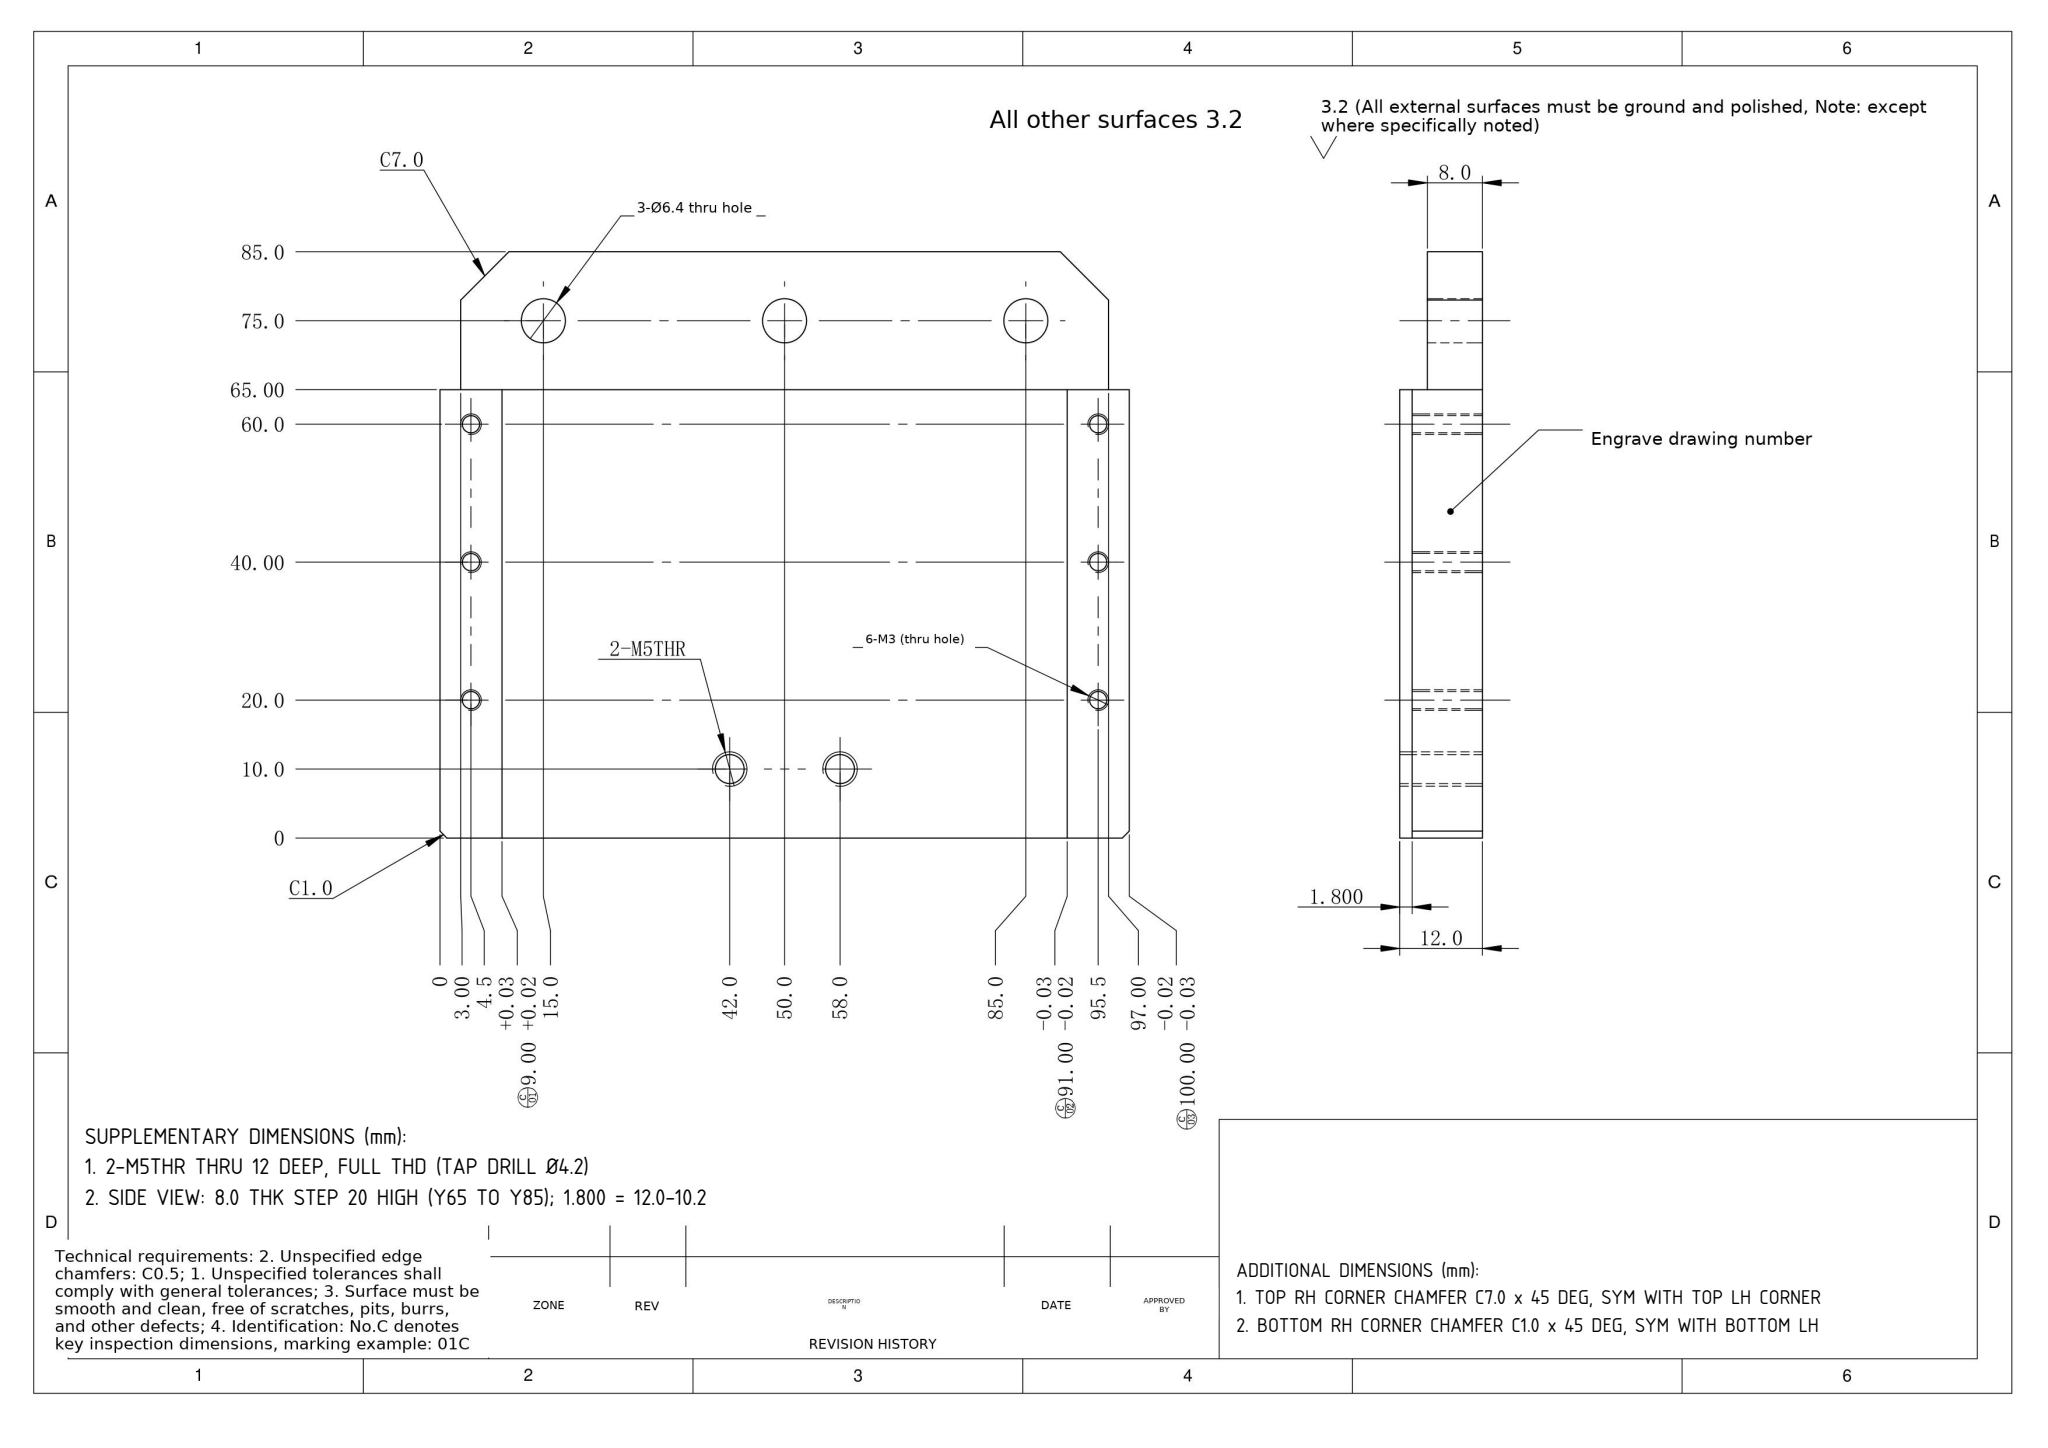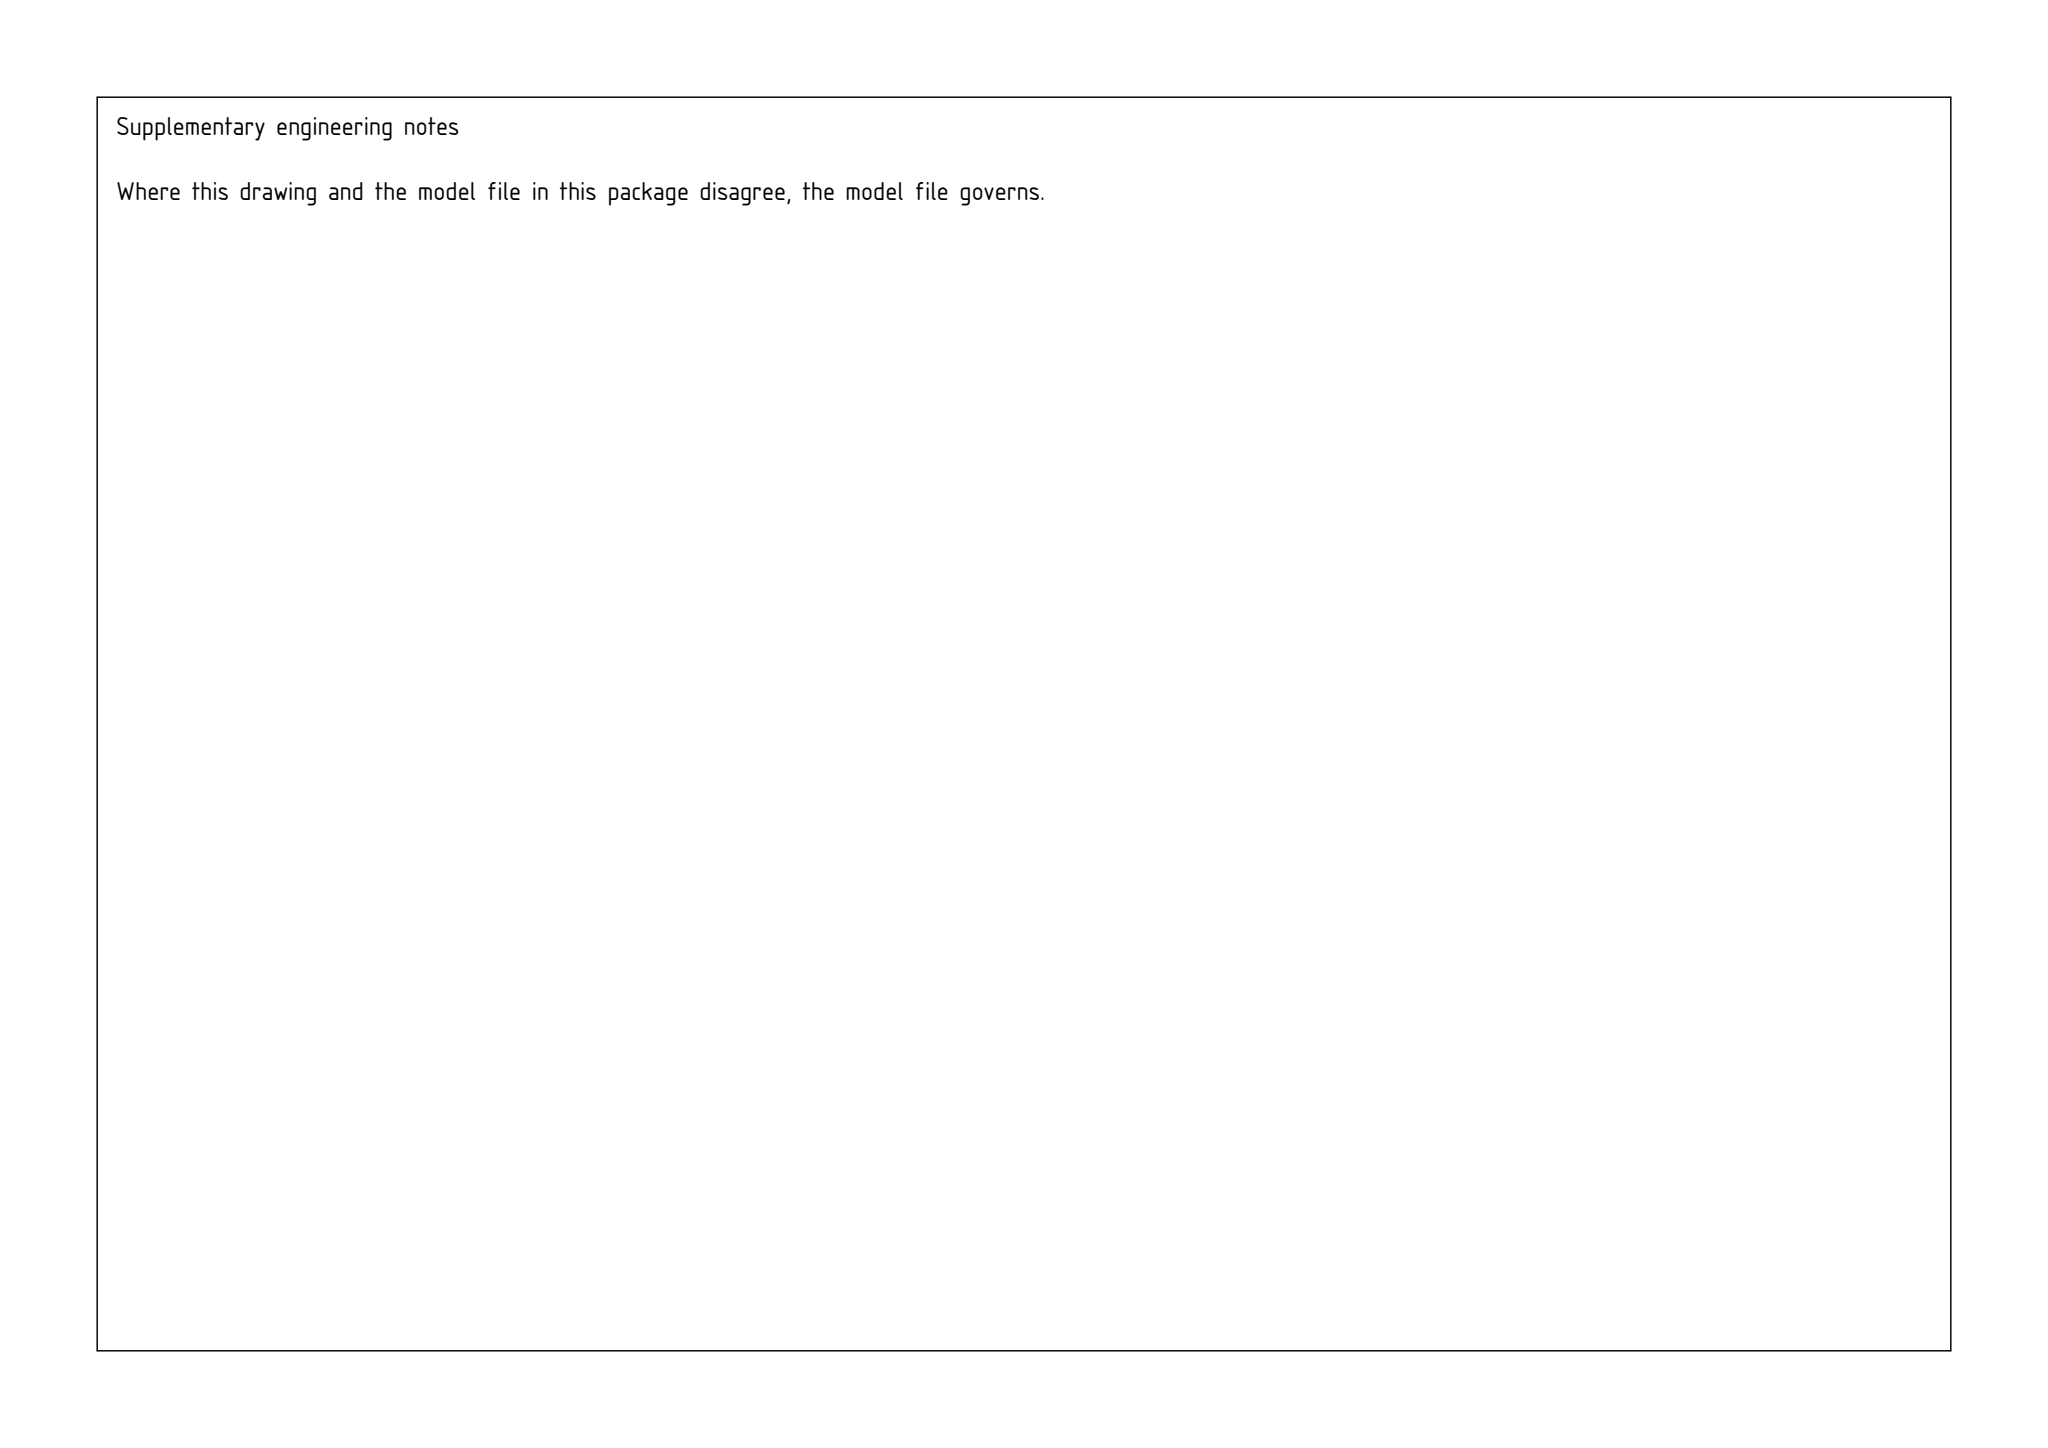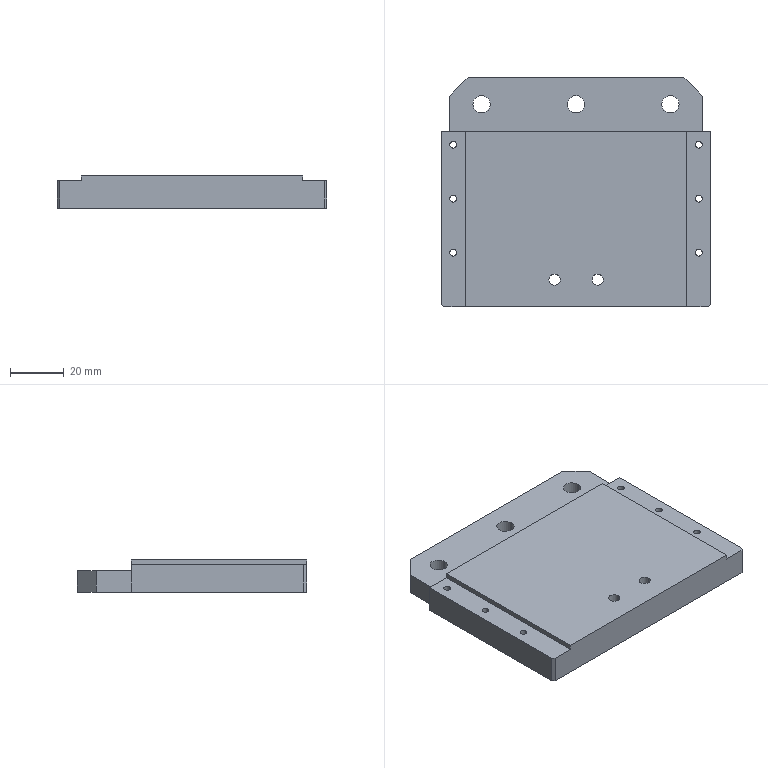Part | SolidWorks | mm | 1 solid | 40 faces | box 100 x 85 x 12 mm | volume 89127 mm3 | cylinder 22 | plane 18 | commonest cylinder face diameters 2.5 x12 6.4 x6 4.2 x4
build123d program:
from build123d import *

# Parameters (mm, degrees)
SKETCH1_W                  = 100
SKETCH1_H                  = 85
BOSS_EXTRUDE1_DEPTH        = 12
SKETCH2_W                  = 9
SKETCH2_H                  = 85
CUT_EXTRUDE1_DEPTH         = 1.8
SKETCH3_W                  = 100
SKETCH3_H                  = 20
CUT_EXTRUDE2_DEPTH         = 4
CHAMFER1_SIZE              = 10
F_5_4_5_4_DIAMETER_HOLE3_D = 5.4
LPATTERN2_COUNT            = 3
LPATTERN2_PITCH            = 35
M3_TAPPED_HOLE1_D          = 2.5
LPATTERN3_COUNT            = 3
LPATTERN3_PITCH            = 20
MIRROR1_COPY_1_D           = 2.5
MIRROR1_COPY_2_D           = 2.5
CHAMFER2_SIZE              = 1
M5_TAPPED_HOLE1_D          = 4.2
CUT_EXTRUDE3_DEPTH         = 10
MOVE_FACE1_BY              = 0.5
MOVE_FACE1_2_BY            = 0.5
MOVE_FACE1_3_BY            = 0.5


with BuildPart() as part:
    # Sketch1 → Boss-Extrude1 (new body)
    with BuildSketch(Plane.XY):
        with Locations((50, 42.5)):
            Rectangle(SKETCH1_W, SKETCH1_H)
    extrude(amount=BOSS_EXTRUDE1_DEPTH)

    # Sketch2 → Cut-Extrude1 (cut)
    with BuildSketch(Plane.XY.offset(12)):
        with Locations((4.5, 42.5)):
            Rectangle(SKETCH2_W, SKETCH2_H)
        with Locations((95.5, 42.5)):
            Rectangle(SKETCH2_W, SKETCH2_H)
    extrude(amount=-CUT_EXTRUDE1_DEPTH, mode=Mode.SUBTRACT)

    # Sketch3 → Cut-Extrude2 (cut)
    with BuildSketch(Plane.XY.offset(12)):
        with Locations((50, 75)):
            Rectangle(SKETCH3_W, SKETCH3_H)
    extrude(amount=-CUT_EXTRUDE2_DEPTH, mode=Mode.SUBTRACT)

    # Chamfer1
    chamfer1_edges = [part.edges().sort_by_distance(p)[0] for p in [
        (100, 85, 4),
        (0, 85, 4),
    ]]
    chamfer(chamfer1_edges, length=CHAMFER1_SIZE)

    # 5.4 _5.4_ Diameter Hole3 (through all)
    with Locations(Plane(origin=(0, 0, 0), x_dir=(-1, 0, 0), z_dir=(0, 0, -1))):
        with Locations((-15, 75)):
            f_5_4_5_4_diameter_hole3 = Hole(F_5_4_5_4_DIAMETER_HOLE3_D / 2)

    # LPattern2: 5.4 _5.4_ Diameter Hole3 ×3
    with Locations(*[(i * LPATTERN2_PITCH, 0, 0) for i in range(1, LPATTERN2_COUNT)]):
        add(f_5_4_5_4_diameter_hole3, mode=Mode.SUBTRACT)

    # M3 Tapped Hole1 (through all)
    with Locations(Plane.XY.offset(10.2)):
        with Locations((95.5, 60)):
            m3_tapped_hole1 = Hole(M3_TAPPED_HOLE1_D / 2)

    # LPattern3: M3 Tapped Hole1 ×3
    with Locations(*[(0, -i * LPATTERN3_PITCH, 0) for i in range(1, LPATTERN3_COUNT)]):
        add(m3_tapped_hole1, mode=Mode.SUBTRACT)

    # Mirror1: M3 Tapped Hole1 across plane
    add(m3_tapped_hole1.mirror(Plane(origin=(50, 0, 0), x_dir=(0, 0, 1), z_dir=(1, 0, 0))), mode=Mode.SUBTRACT)

    # Mirror1 copy 1 (through all)
    with Locations(Plane(origin=(100, -20, 10.2), x_dir=(-1, 0, 0), z_dir=(0, 0, 1))):
        with Locations((95.5, -60)):
            Hole(MIRROR1_COPY_1_D / 2)

    # Mirror1 copy 2 (through all)
    with Locations(Plane(origin=(100, -40, 10.2), x_dir=(-1, 0, 0), z_dir=(0, 0, 1))):
        with Locations((95.5, -60)):
            Hole(MIRROR1_COPY_2_D / 2)

    # Chamfer2
    chamfer2_edges = [part.edges().sort_by_distance(p)[0] for p in [
        (0, 0, 5.1),
        (100, 0, 5.1),
    ]]
    chamfer(chamfer2_edges, length=CHAMFER2_SIZE)

    # M5 Tapped Hole1 (through all)
    with Locations(Plane(origin=(42.039, 10, 12), x_dir=(1, 0, 0), z_dir=(0, 0, 1))):
        with Locations((0, 0), (16, 0)):
            Hole(M5_TAPPED_HOLE1_D / 2)

    # Sketch13 → Cut-Extrude3 (cut)
    with BuildSketch(Plane.XY.offset(8)):
        Polygon((0, 75), (0, 65), (3, 65), (3, 78), align=None)
        Polygon((97, 83), (97, 78), (100, 75), (100, 85), (97, 85), align=None)
        Polygon((97, 78), (97, 65), (100, 65), (100, 75), align=None)
    extrude(amount=-CUT_EXTRUDE3_DEPTH, mode=Mode.SUBTRACT)

    # Move Face1: a curved face moved inward by 0.5
    add(Solid.thicken(part.faces().sort_by_distance((12.3, 75, 4))[0], -MOVE_FACE1_BY), mode=Mode.SUBTRACT)

    # Move Face1 2: a curved face moved inward by 0.5
    add(Solid.thicken(part.faces().sort_by_distance((47.3, 75, 4))[0], -MOVE_FACE1_2_BY), mode=Mode.SUBTRACT)

    # Move Face1 3: a curved face moved inward by 0.5
    add(Solid.thicken(part.faces().sort_by_distance((82.3, 75, 4))[0], -MOVE_FACE1_3_BY), mode=Mode.SUBTRACT)


solid = part.part